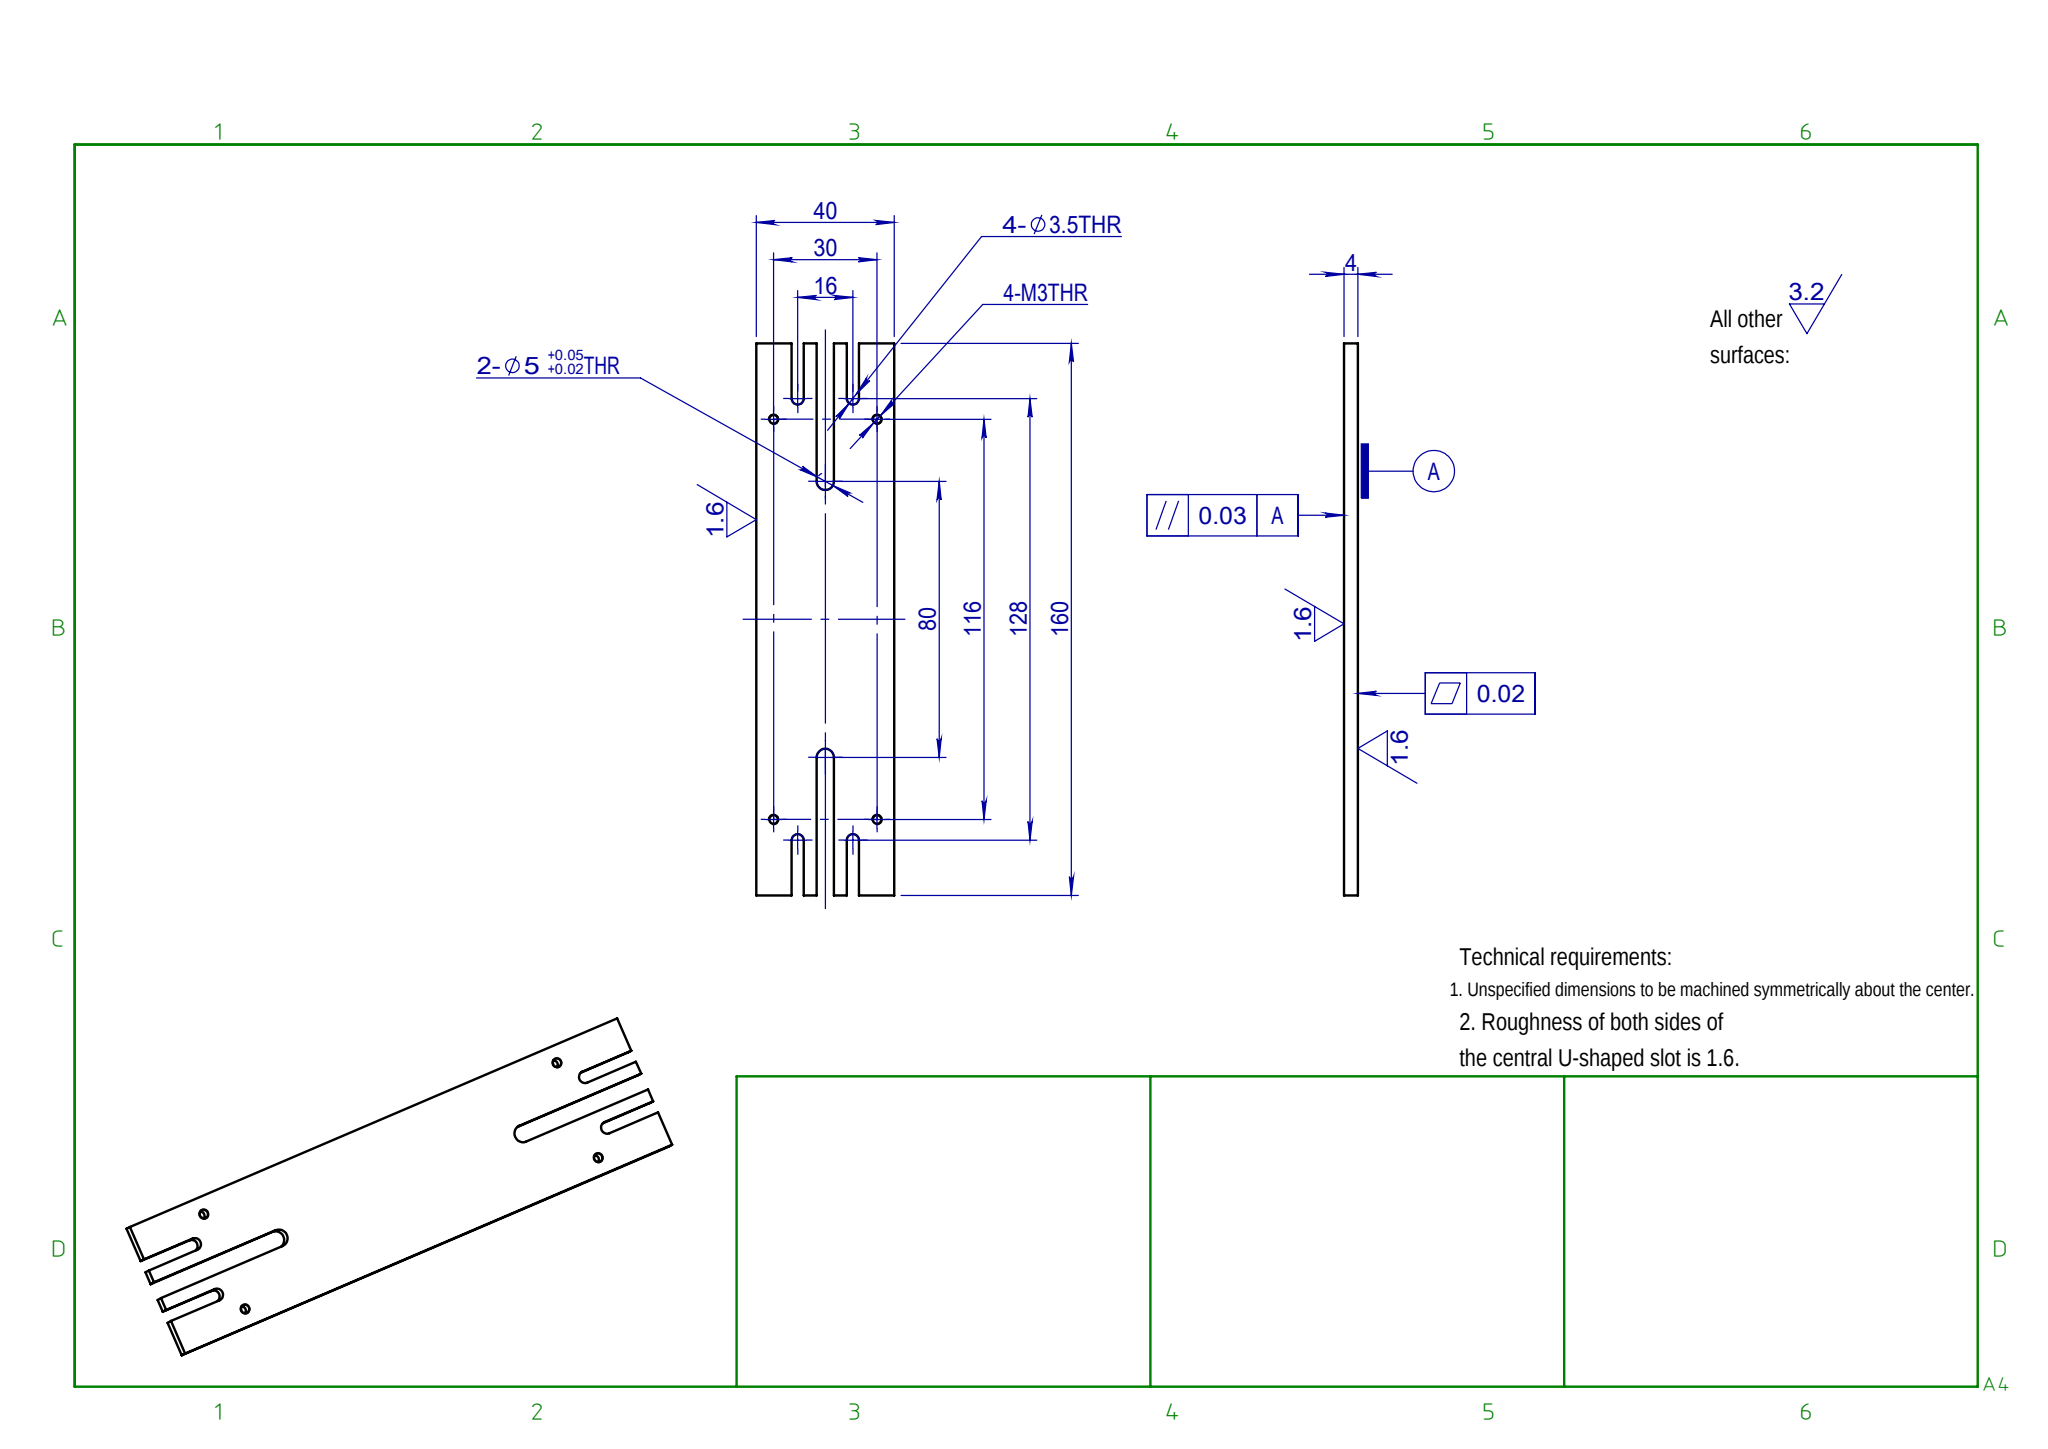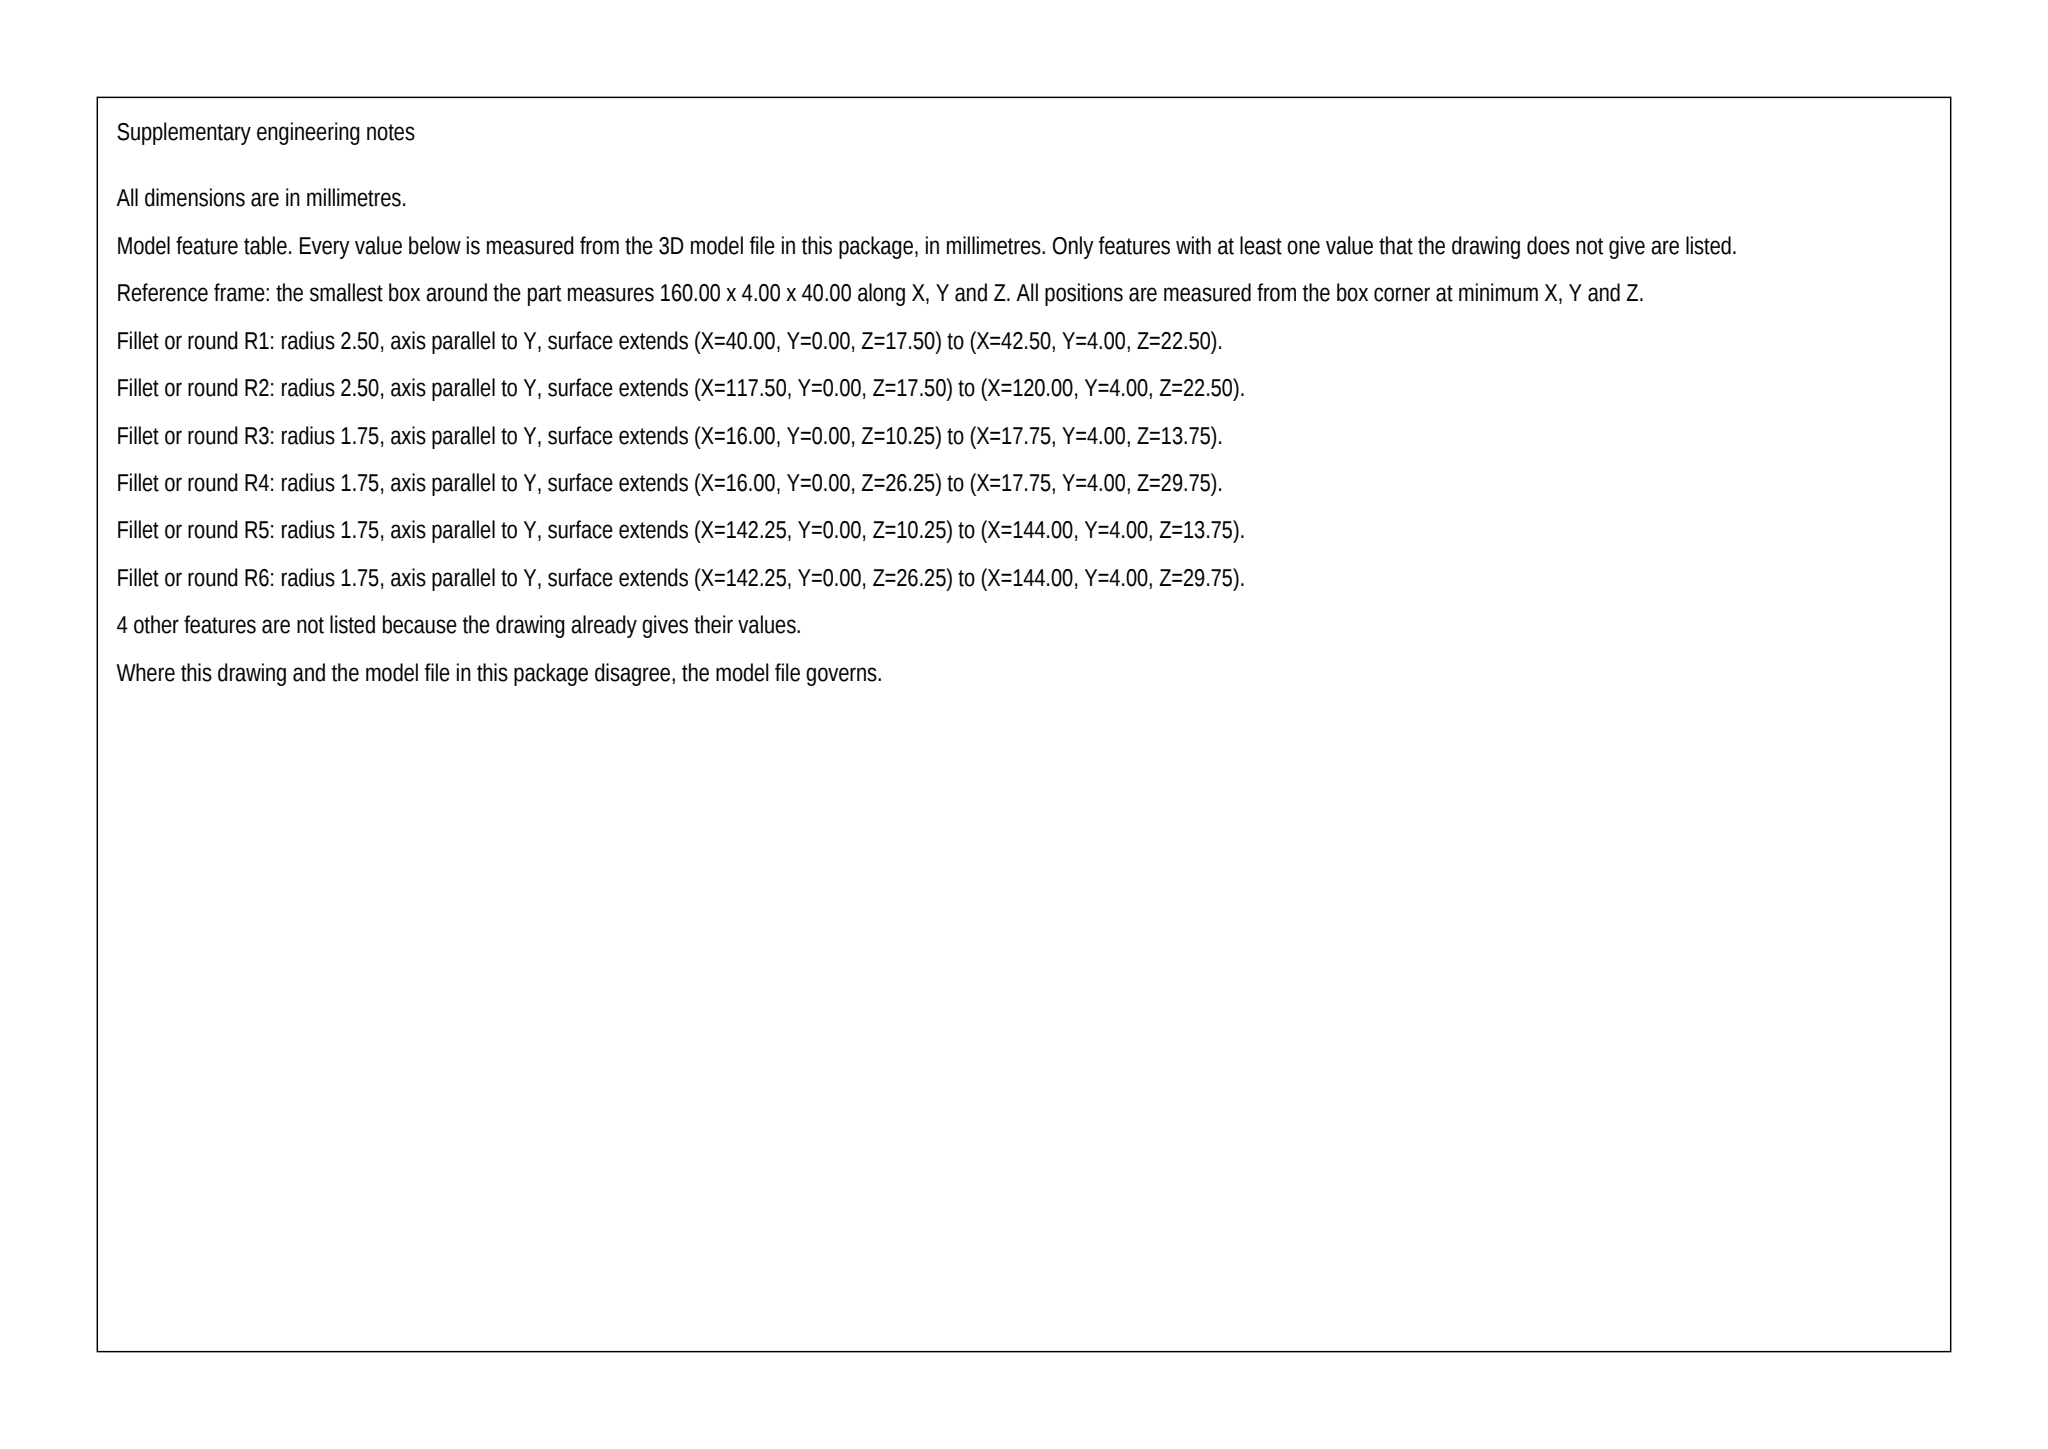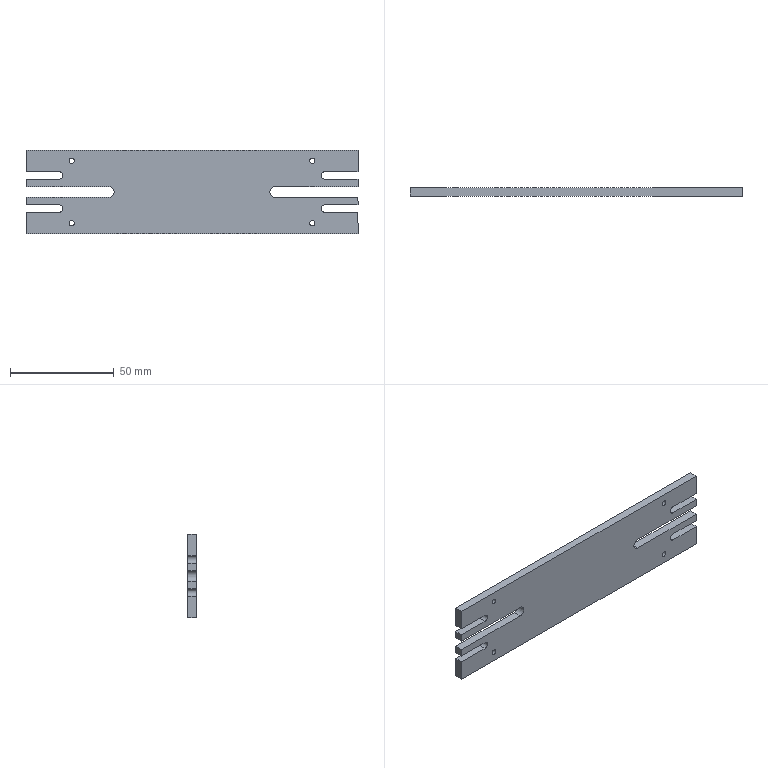Part | SolidWorks | mm | material Plain Carbon Steel | 1 solid | 38 faces | box 160 x 4 x 40 mm | volume 22870 mm3 | plane 24 | cylinder 14 | commonest cylinder face diameters 2.5 x8 3.5 x4 5 x2
build123d program:
from build123d import *

# Parameters (mm, degrees)
SKETCH1_W             = 160
SKETCH1_H             = 40
EXTRUDE1_DEPTH        = 4
M3_TAPPED_HOLE1_D     = 2.5
M3_TAPPED_HOLE1_DEPTH = 8.5
M3_TAPPED_HOLE1_TIP   = 0.7511
CUT_EXTRUDE1_DEPTH    = 83.559
CUT_EXTRUDE2_DEPTH    = 83.559


with BuildPart() as part:
    # Sketch1 → Extrude1 (new body)
    with BuildSketch(Plane(origin=(0, 0, 0), x_dir=(1, 0, 0), z_dir=(0, 1, 0))):
        Rectangle(SKETCH1_W, SKETCH1_H)
    extrude(amount=EXTRUDE1_DEPTH)

    # M3 Tapped Hole1
    with Locations(Plane(origin=(0, 4, 0), x_dir=(1, 0, 0), z_dir=(0, 1, 0))):
        with Locations((-58, -15), (-58, 15), (58, -15), (58, 15)):
            Hole(M3_TAPPED_HOLE1_D / 2, depth=M3_TAPPED_HOLE1_DEPTH)
            with Locations((0, 0, -(M3_TAPPED_HOLE1_DEPTH + M3_TAPPED_HOLE1_TIP / 2))):  # 118° drill point
                Cone(0, M3_TAPPED_HOLE1_D / 2, M3_TAPPED_HOLE1_TIP, mode=Mode.SUBTRACT)

    # Sketch4 → Cut-Extrude1 (cut, through all)
    with BuildSketch(Plane(origin=(0, 4, 0), x_dir=(1, 0, 0), z_dir=(0, 1, 0))):
        with BuildLine():
            Line((-80, -2.5), (-80, 2.5))
            Line((-80, 2.5), (-40, 2.5))
            ThreePointArc((-40, 2.5), (-37.5, 0), (-40, -2.5))
            Line((-40, -2.5), (-80, -2.5))
        make_face()
        with BuildLine():
            Line((40, -2.5), (80, -2.5))
            Line((80, -2.5), (80, 2.5))
            Line((80, 2.5), (40, 2.5))
            ThreePointArc((40, 2.5), (37.5, 0), (40, -2.5))
        make_face()
    extrude(amount=-CUT_EXTRUDE1_DEPTH, mode=Mode.SUBTRACT)

    # Sketch5 → Cut-Extrude2 (cut, through all)
    with BuildSketch(Plane(origin=(0, 4, 0), x_dir=(1, 0, 0), z_dir=(0, 1, 0))):
        with BuildLine():
            Line((-64, 9.75), (-80, 9.75))
            Line((-80, 9.75), (-80, 6.25))
            Line((-80, 6.25), (-64, 6.25))
            ThreePointArc((-64, 6.25), (-62.25, 8), (-64, 9.75))
        make_face()
        with BuildLine():
            Line((-64, -6.25), (-80, -6.25))
            Line((-80, -6.25), (-80, -9.75))
            Line((-80, -9.75), (-64, -9.75))
            ThreePointArc((-64, -9.75), (-62.25, -8), (-64, -6.25))
        make_face()
        with BuildLine():
            Line((64, 9.75), (80, 9.75))
            Line((80, 9.75), (80, 6.25))
            Line((80, 6.25), (64, 6.25))
            ThreePointArc((64, 6.25), (62.25, 8), (64, 9.75))
        make_face()
        with BuildLine():
            Line((64, -6.25), (80, -6.25))
            Line((80, -6.25), (80, -9.75))
            Line((80, -9.75), (64, -9.75))
            ThreePointArc((64, -9.75), (62.25, -8), (64, -6.25))
        make_face()
    extrude(amount=-CUT_EXTRUDE2_DEPTH, mode=Mode.SUBTRACT)


solid = part.part